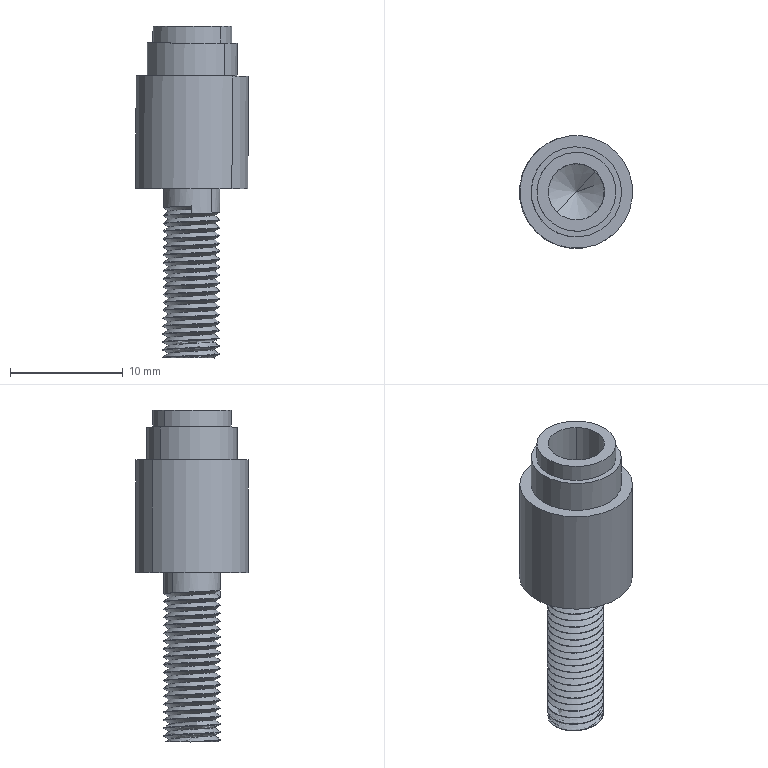Component | SolidWorks | Light-1_Screw1-1 | 1 solid | 57 faces | volume 1032 mm3 | cylinder 46 | plane 6 | spline 3 | cone 2 | commonest cylinder face diameters 5 x40 8 x2 10 x2 7 x2